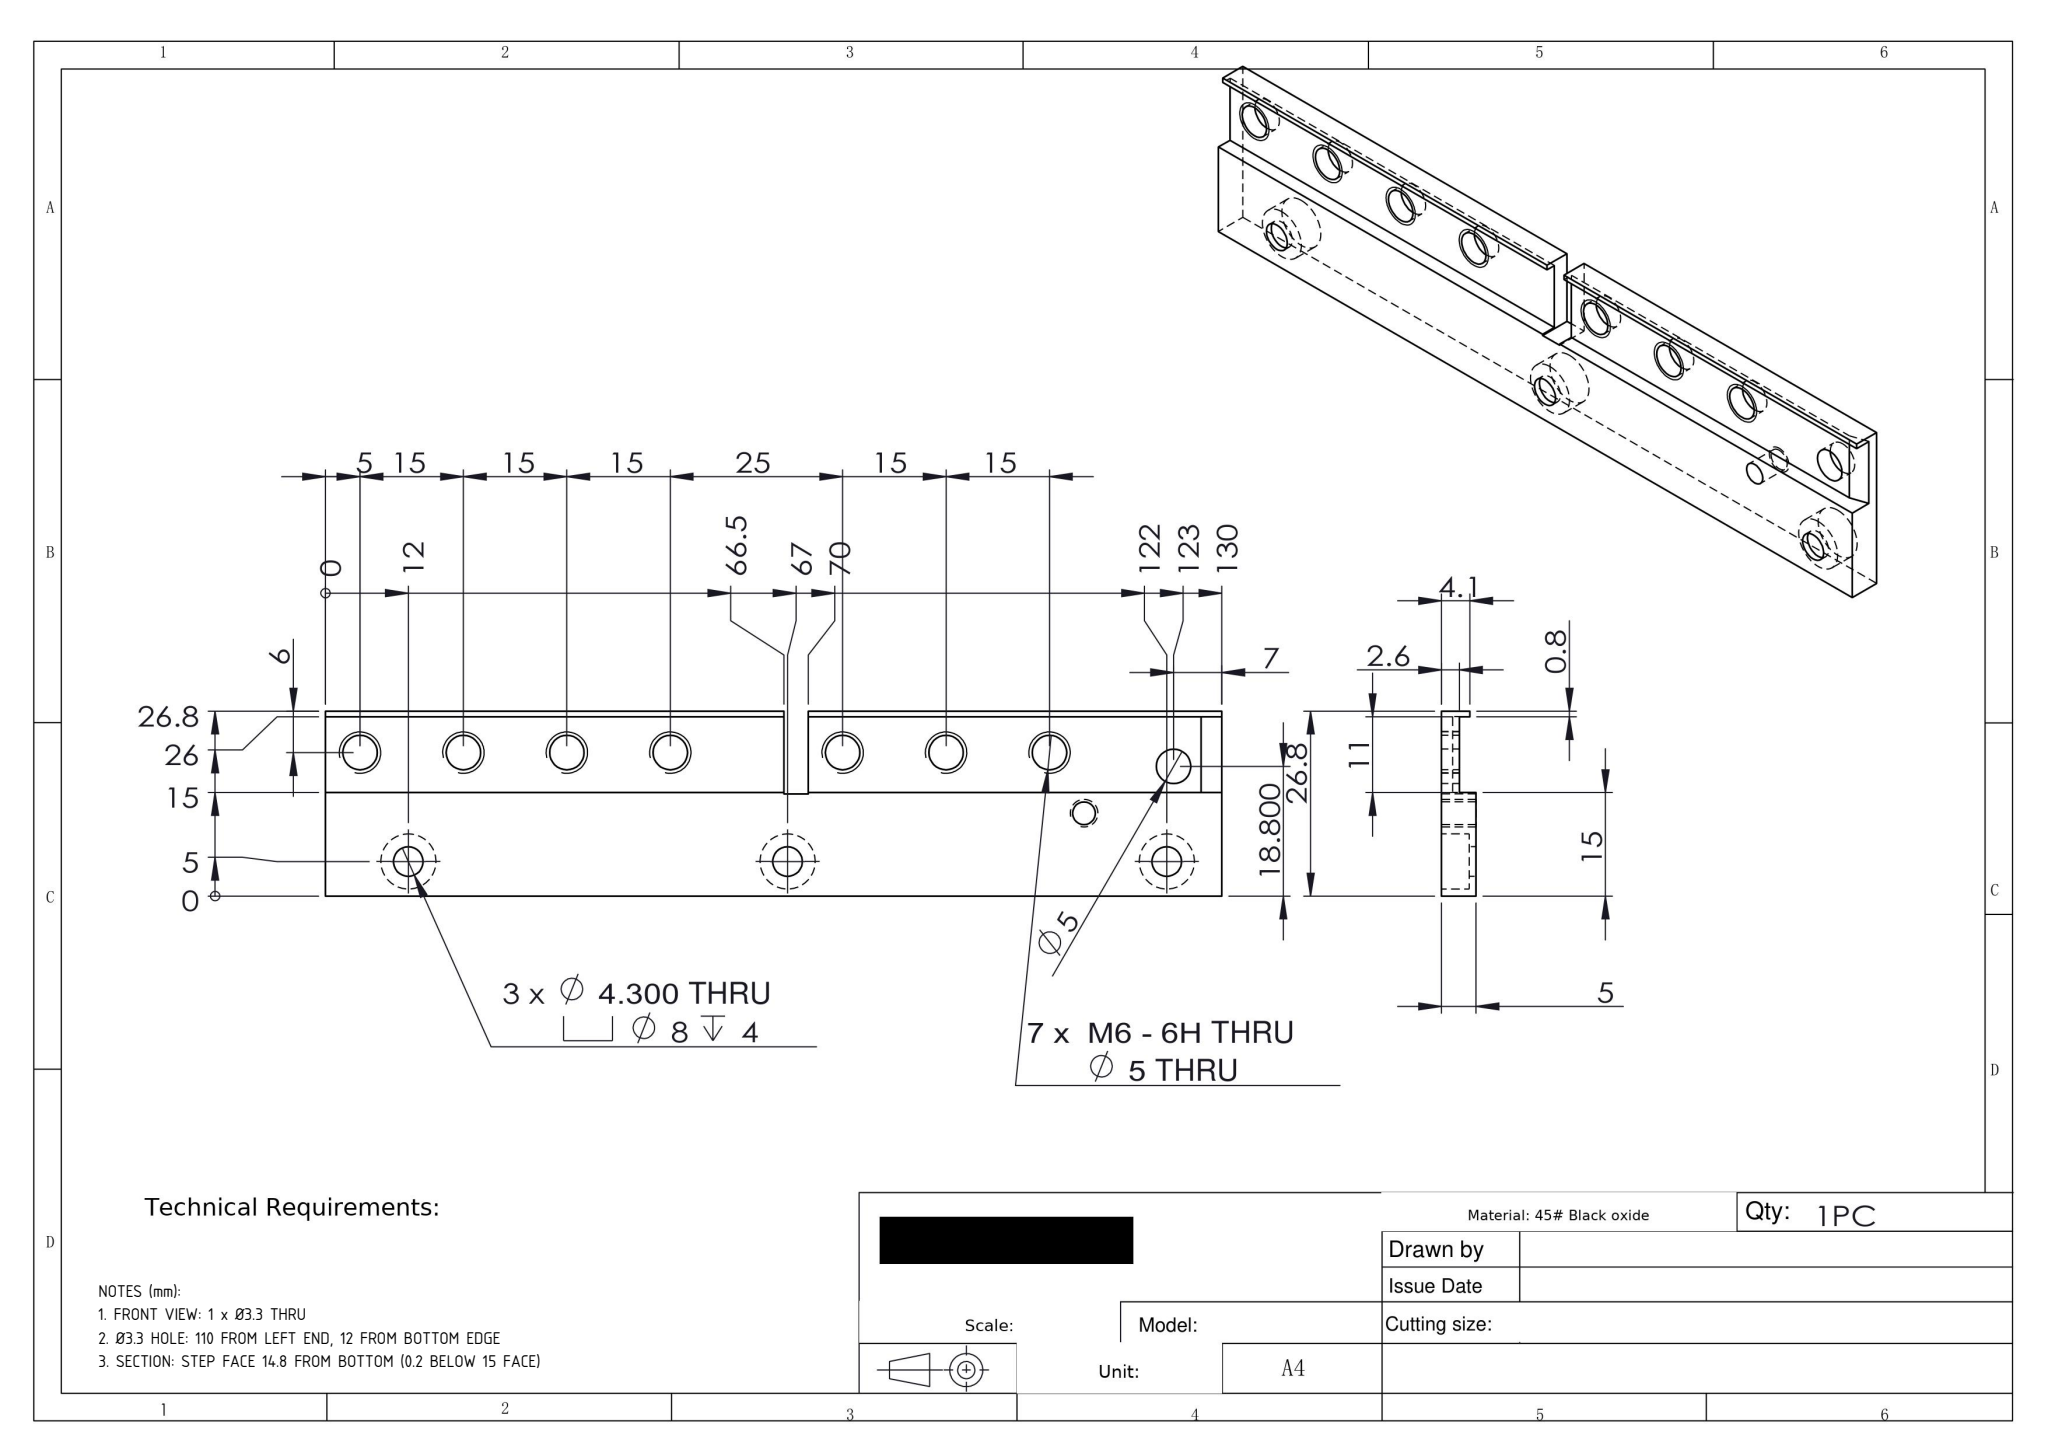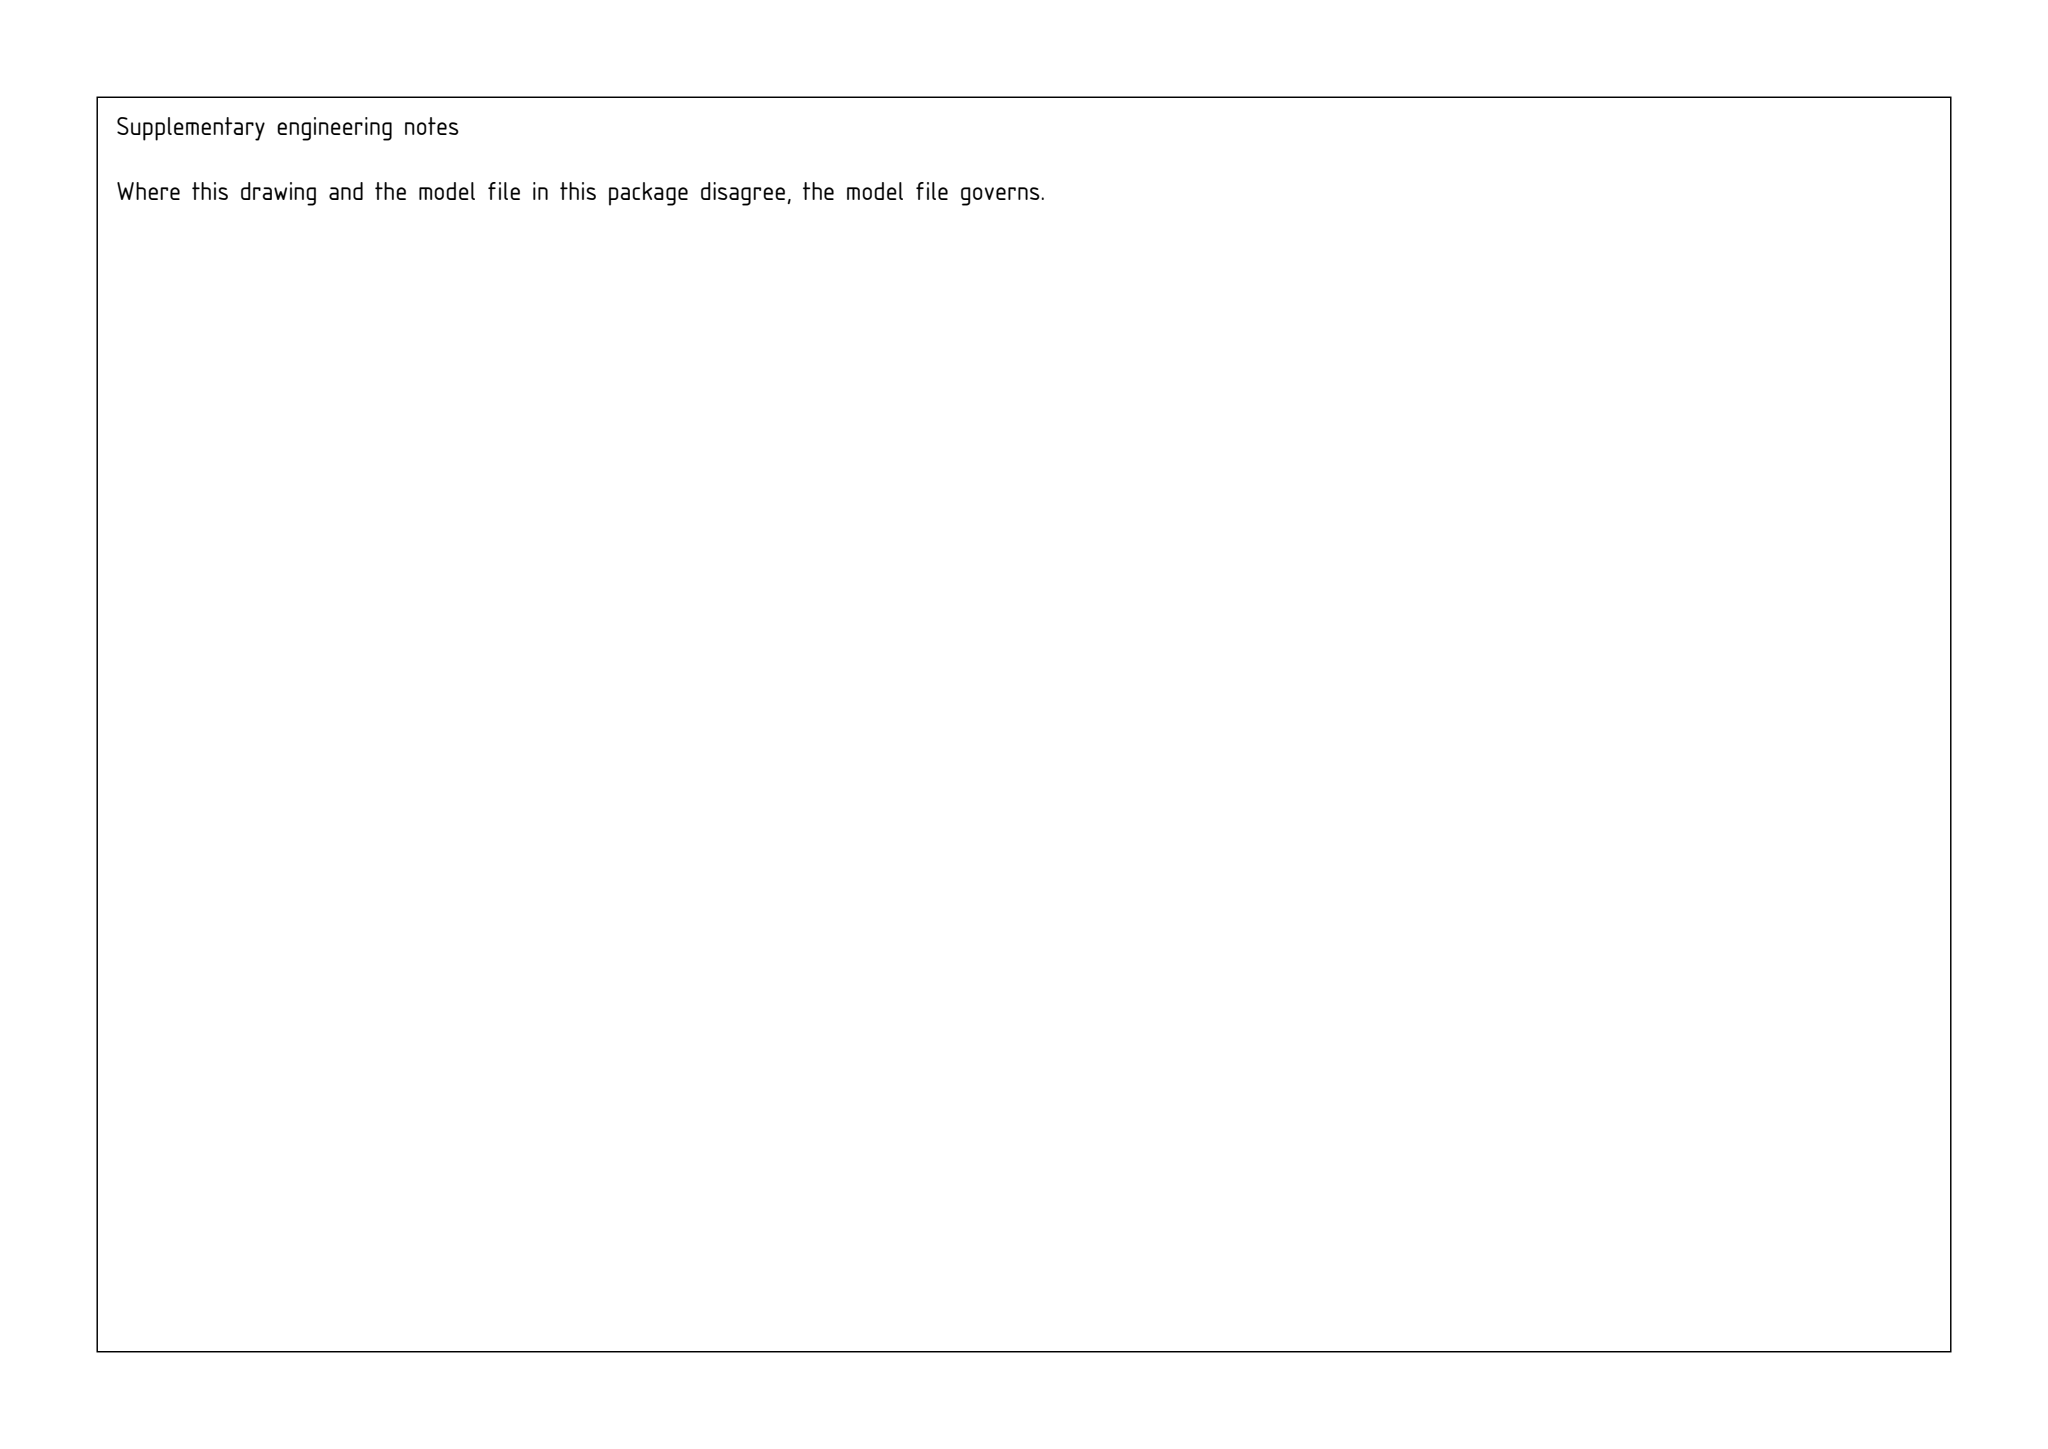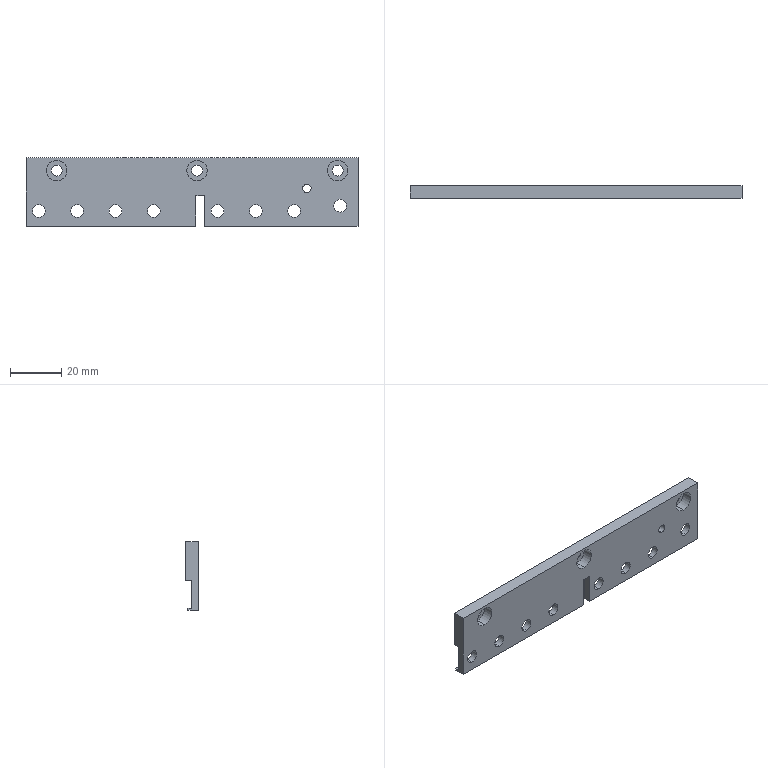Part | SolidWorks | mm | 1 solid | 52 faces | box 130 x 5 x 26.8 mm | volume 12665 mm3 | cylinder 30 | plane 22 | commonest cylinder face diameters 5 x16 8 x6 4.3 x6 3.3 x2
Drawing notes:
FRONT VIEW: 1 x Ø3.3 THRU | from the solid: cylinder dia 3.3, axis y, length 5.0 = full 5 thk, at x=110, z=14.8
Ø3.3 HOLE: 110 FROM LEFT END, 12 FROM BOTTOM EDGE | from the solid: 3.3 hole pos [110, -, 14.8]; bbox z 26.8 so 26.8-14.8=12 up from bottom face
SECTION: STEP FACE 14.8 FROM BOTTOM (0.2 BELOW 15 FACE) | from the solid: z-plane offset 12.0 (single) vs 11.8 pair; 26.8-12.0=14.8, 26.8-11.8=15.0
build123d program:
from build123d import *

# Parameters (mm, degrees)
SKETCH1_W                                       = 130
SKETCH1_H                                       = 26.8
BOSS_EXTRUDE1_DEPTH                             = 5
SKETCH2_W                                       = 130
SKETCH2_H                                       = 11
CUT_EXTRUDE1_DEPTH                              = 2.4
M4_HEX_SOCKET_HEAD_CAP_SCREW_CBORE1_D           = 4.3
M4_HEX_SOCKET_HEAD_CAP_SCREW_CBORE1_CBORE_D     = 8
M4_HEX_SOCKET_HEAD_CAP_SCREW_CBORE1_CBORE_DEPTH = 4
SKETCH5_W                                       = 130
SKETCH5_H                                       = 0.8
CUT_EXTRUDE2_DEPTH                              = 0.9
SKETCH6_W                                       = 3.5
SKETCH6_H                                       = 12
CUT_EXTRUDE3_DEPTH                              = 10
SKETCH7_R                                       = 2.5
CUT_EXTRUDE4_DEPTH                              = 10
CHAMFER2_SIZE                                   = 1
CHAMFER2_SIZE2                                  = 3
M4_TAPPED_HOLE1_D                               = 3.3
M4_TAPPED_HOLE1_DEPTH                           = 10.1
M4_TAPPED_HOLE1_TIP                             = 0.9914
M6_TAPPED_HOLE1_D                               = 5


with BuildPart() as part:
    # Sketch1 → Boss-Extrude1 (new body)
    with BuildSketch(Plane(origin=(0, 0, 0), x_dir=(1, 0, 0), z_dir=(0, 1, 0))):
        with Locations((65, 13.4)):
            Rectangle(SKETCH1_W, SKETCH1_H)
    extrude(amount=BOSS_EXTRUDE1_DEPTH)

    # Sketch2 → Cut-Extrude1 (cut)
    with BuildSketch(Plane(origin=(0, 5, 0), x_dir=(1, 0, 0), z_dir=(0, 1, 0))):
        with Locations((65, 20.5)):
            Rectangle(SKETCH2_W, SKETCH2_H)
    extrude(amount=-CUT_EXTRUDE1_DEPTH, mode=Mode.SUBTRACT)

    # M4 Hex Socket Head Cap Screw CBORE1 (through all)
    with Locations(Plane.XZ):
        with Locations((12, -5), (122, -5), (67, -5)):
            CounterBoreHole(M4_HEX_SOCKET_HEAD_CAP_SCREW_CBORE1_D / 2, M4_HEX_SOCKET_HEAD_CAP_SCREW_CBORE1_CBORE_D / 2, M4_HEX_SOCKET_HEAD_CAP_SCREW_CBORE1_CBORE_DEPTH)

    # Sketch5 → Cut-Extrude2 (cut)
    with BuildSketch(Plane(origin=(0, 5, 0), x_dir=(1, 0, 0), z_dir=(0, 1, 0))):
        with Locations((65, 26.4)):
            Rectangle(SKETCH5_W, SKETCH5_H)
    extrude(amount=-CUT_EXTRUDE2_DEPTH, mode=Mode.SUBTRACT)

    # Sketch6 → Cut-Extrude3 (cut)
    with BuildSketch(Plane.XZ):
        with Locations((68.25, -20.8)):
            Rectangle(SKETCH6_W, SKETCH6_H)
    extrude(amount=-CUT_EXTRUDE3_DEPTH, mode=Mode.SUBTRACT)

    # Sketch7 → Cut-Extrude4 (cut)
    with BuildSketch(Plane(origin=(0, 0, 0), x_dir=(-1, 0, 0), z_dir=(0, -1, 0))):
        with Locations(Location((-123, 18.8, 0), (0, 0, 90))):
            Circle(SKETCH7_R)
    extrude(amount=-CUT_EXTRUDE4_DEPTH, mode=Mode.SUBTRACT)

    # Chamfer2
    chamfer2_edges = [part.edges().sort_by_distance(p)[0] for p in [
        (130, 2.6, -20.5),
    ]]
    chamfer2_side = [part.faces().sort_by_distance(p)[0] for p in [
        (130, 2.165, -11.559),
    ]]
    chamfer(chamfer2_edges, length=CHAMFER2_SIZE, length2=CHAMFER2_SIZE2, reference=chamfer2_side[0])

    # M4 Tapped Hole1
    with Locations(Plane(origin=(110, 0, -12), x_dir=(0, 0, -1), z_dir=(0, -1, 0))):
        with Locations((0, 0)):
            Hole(M4_TAPPED_HOLE1_D / 2, depth=M4_TAPPED_HOLE1_DEPTH)
            with Locations((0, 0, -(M4_TAPPED_HOLE1_DEPTH + M4_TAPPED_HOLE1_TIP / 2))):  # 118° drill point
                Cone(0, M4_TAPPED_HOLE1_D / 2, M4_TAPPED_HOLE1_TIP, mode=Mode.SUBTRACT)

    # M6 Tapped Hole1 (through all)
    with Locations(Plane(origin=(0, 2.6, 0), x_dir=(1, 0, 0), z_dir=(0, 1, 0))):
        with Locations((5, 20.8), (20, 20.8), (35, 20.8), (50, 20.8), (75, 20.8), (90, 20.8), (105, 20.8)):
            Hole(M6_TAPPED_HOLE1_D / 2)


solid = part.part